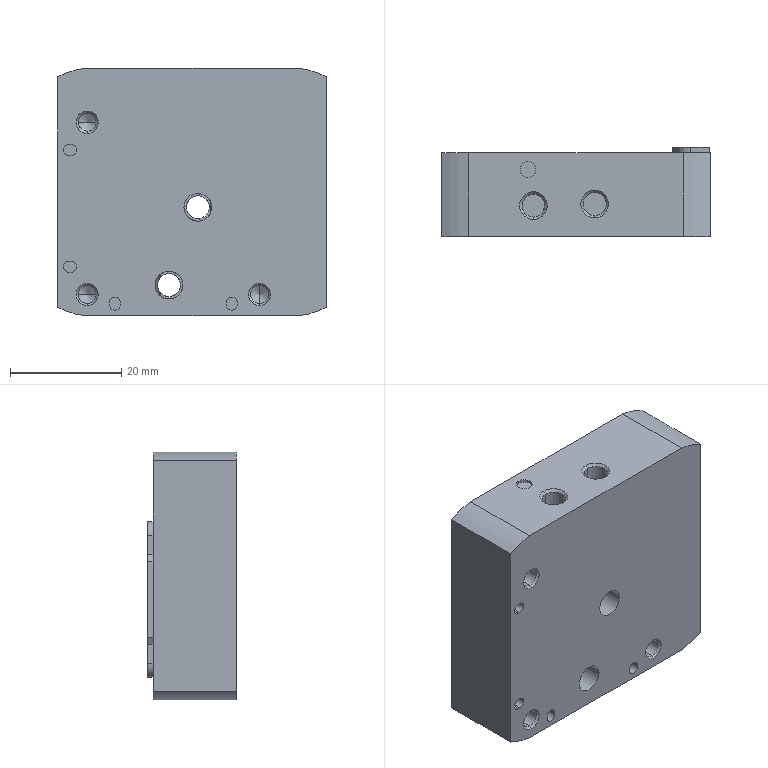Component | SolidWorks | DGC-18-280-G-PPV-A-1_HI_532446 DGC-18-G---(0DR)_1-1 | 1 solid | 114 faces | volume 30427 mm3 | cylinder 48 | plane 46 | cone 20 | commonest cylinder face diameters 5 x14 2 x10 4.134 x8 3.242 x6 4.2 x4 29.667 x4 2.8 x2